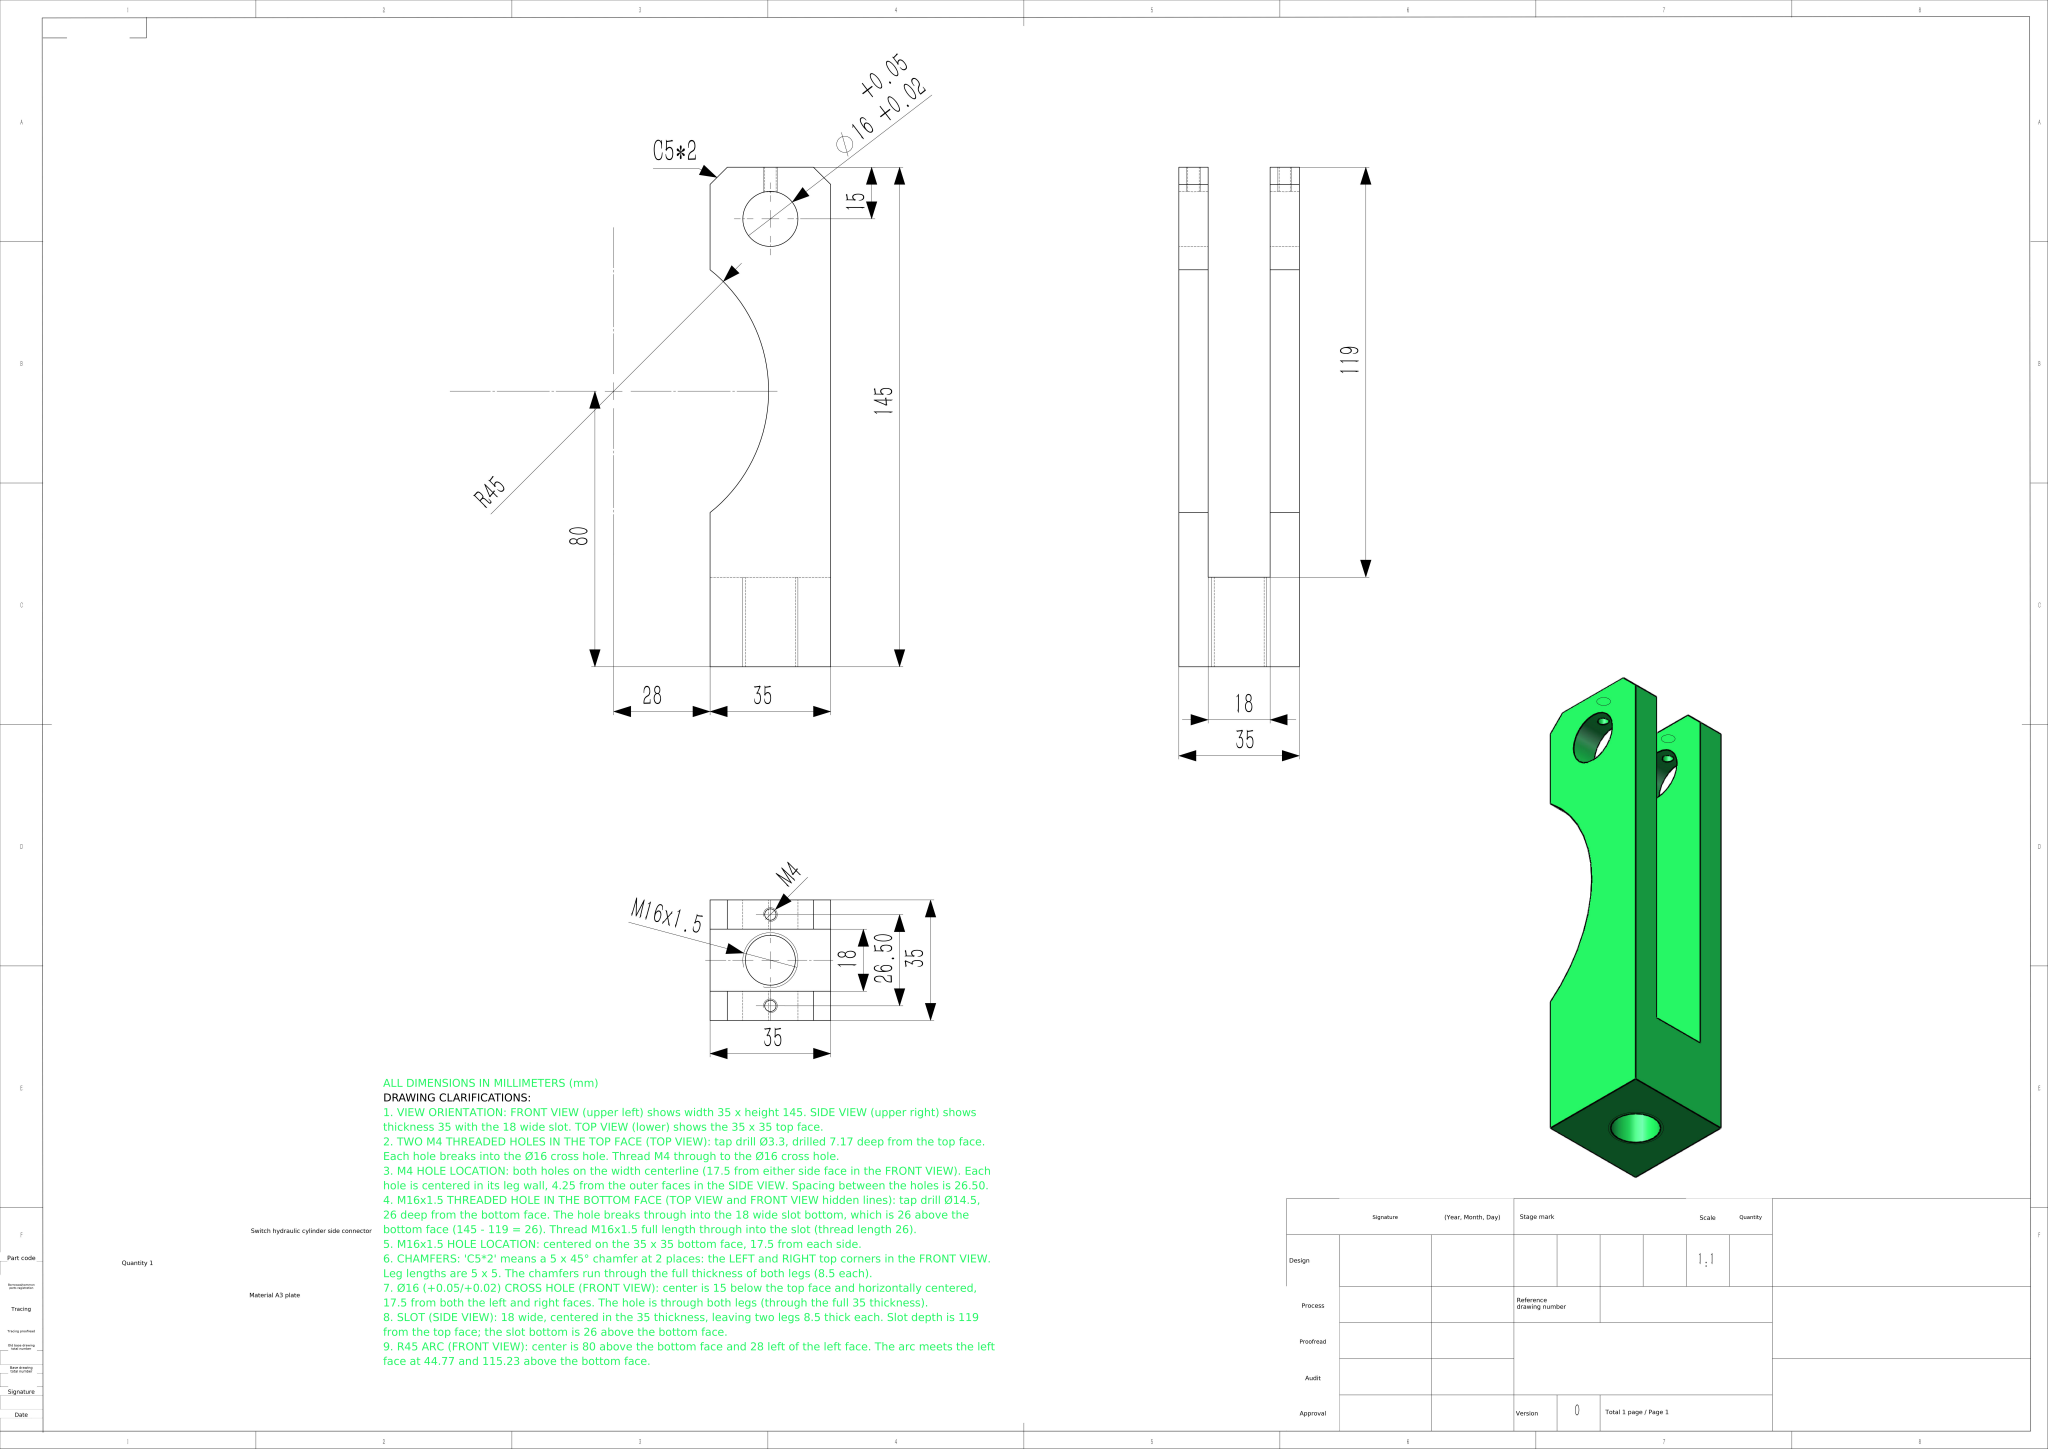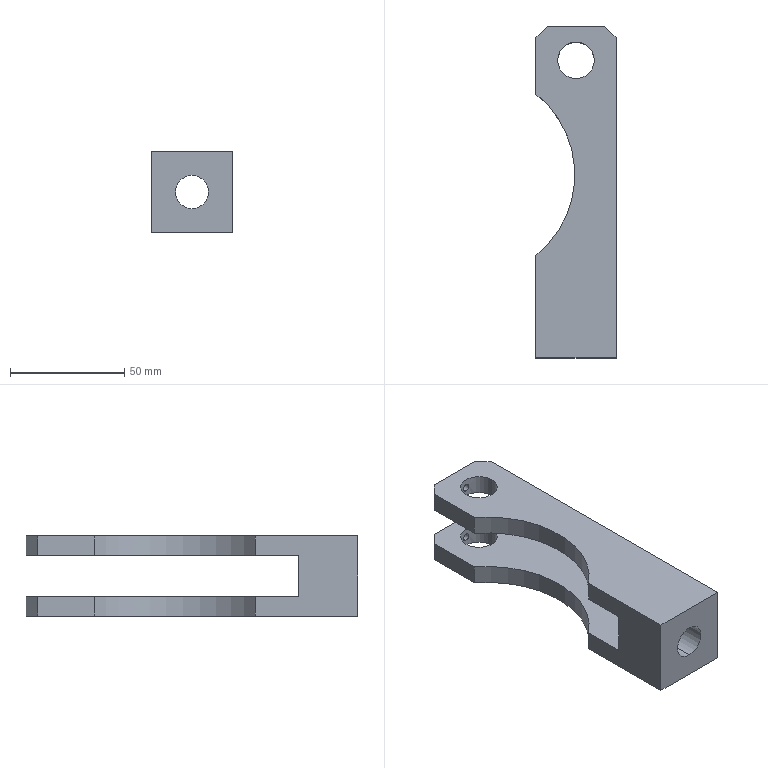Part | NX | mm | Angled Dual-Ear Clevis Bracket | 1 solid | 28 faces | box 35 x 145 x 35 mm | volume 80211 mm3 | plane 16 | cylinder 12 | commonest cylinder face diameters 3.3 x4 16 x4 14.5 x2 90 x2